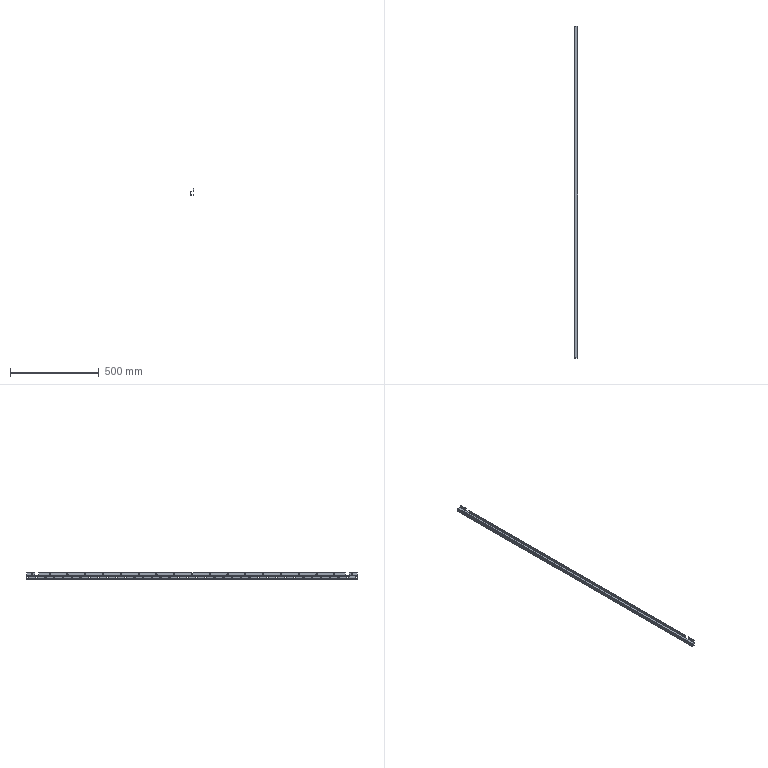Component | SolidWorks | RightFrontDoorAssembly-1_DoorRearVerticalStiffener06-1-2 | 1 solid | 168 faces | volume 119430 mm3 | cylinder 124 | plane 44 | commonest cylinder face diameters 10 x76 7 x38 5 x5 3 x5